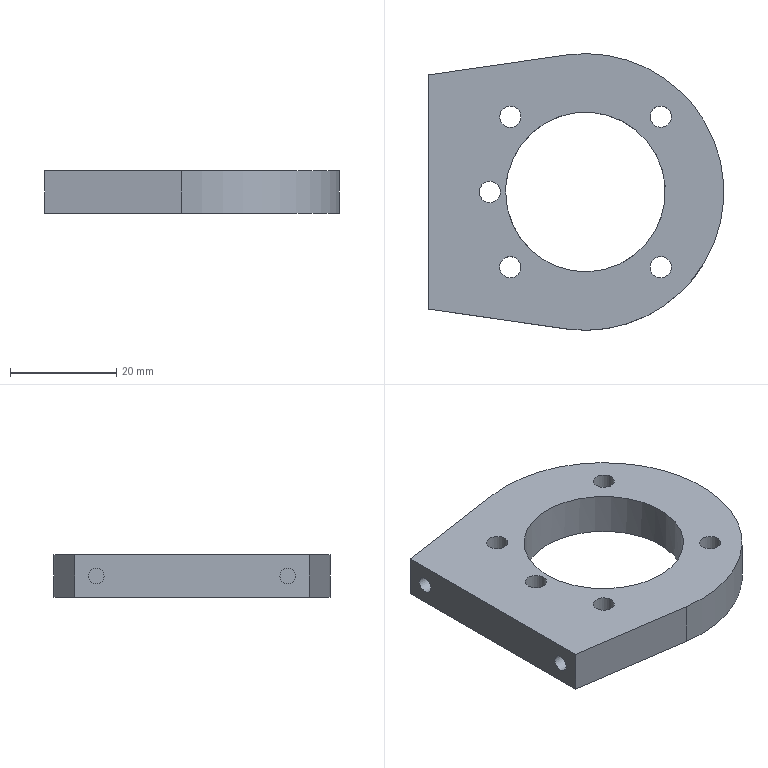Component | NX | 03C__27_2 | 1 solid | 18 faces | volume 13507 mm3 | cylinder 10 | plane 8 | commonest cylinder face diameters 4 x5 3 x2 52 x1 30 x1 8 x1